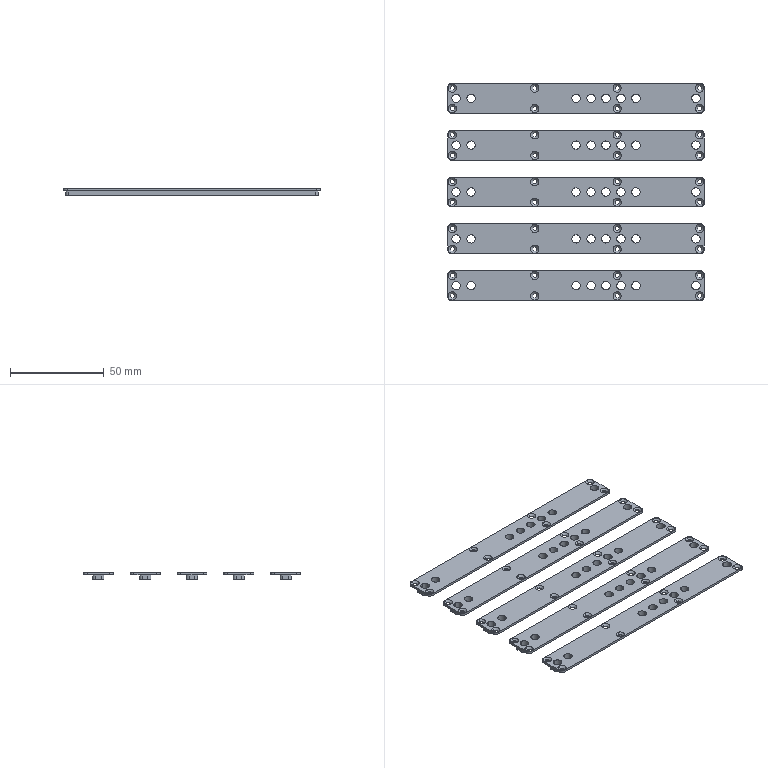CAM job | Mastercam | mm | 8 operations | part box 137 x 116 x 3.5
1. Facing | 8 - 8 平铣刀
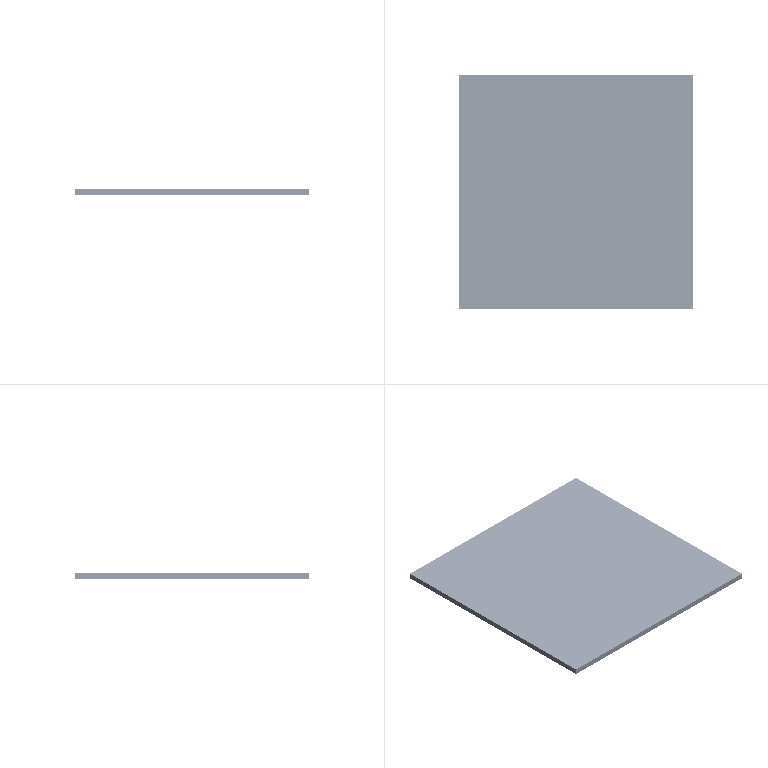2. Contour (Ramp) | 8 - 8 平铣刀
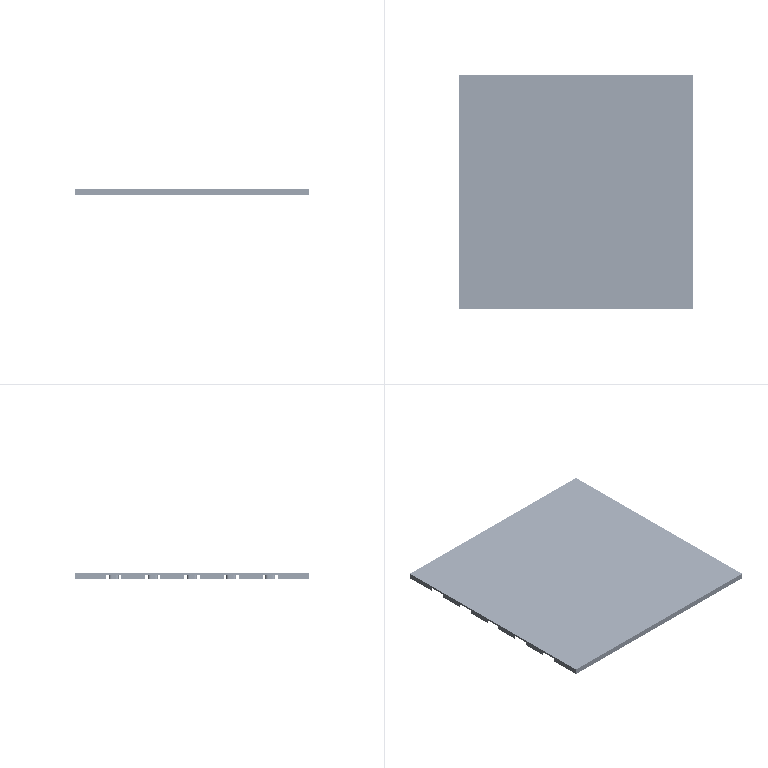3. Contour (2D) | 6 - 6 平铣刀
4. Contour (Ramp) | 3 - 3 平铣刀
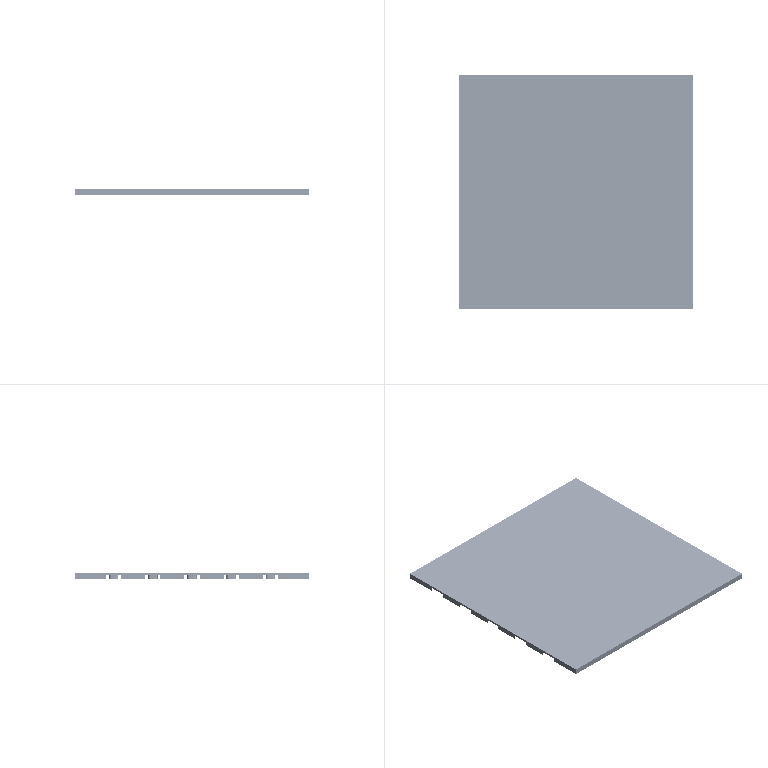5. Drill/Counterbore | 7 - 4 倒角刀
6. Contour (2D chamfer) | 7 - 4 倒角刀
7. Contour (2D chamfer) | 7 - 4 倒角刀
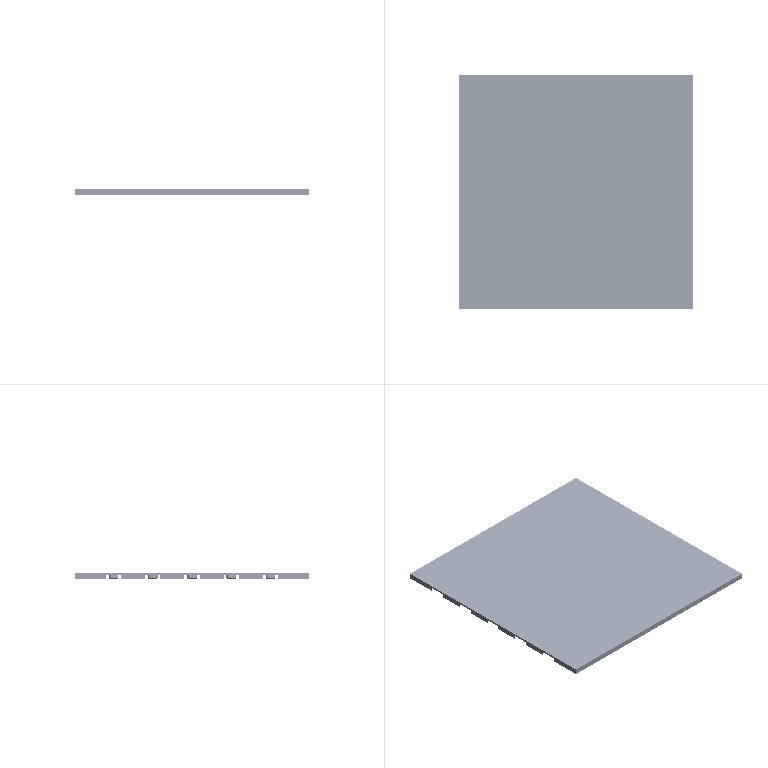8. Contour (2D) | 2 - 2 平铣刀